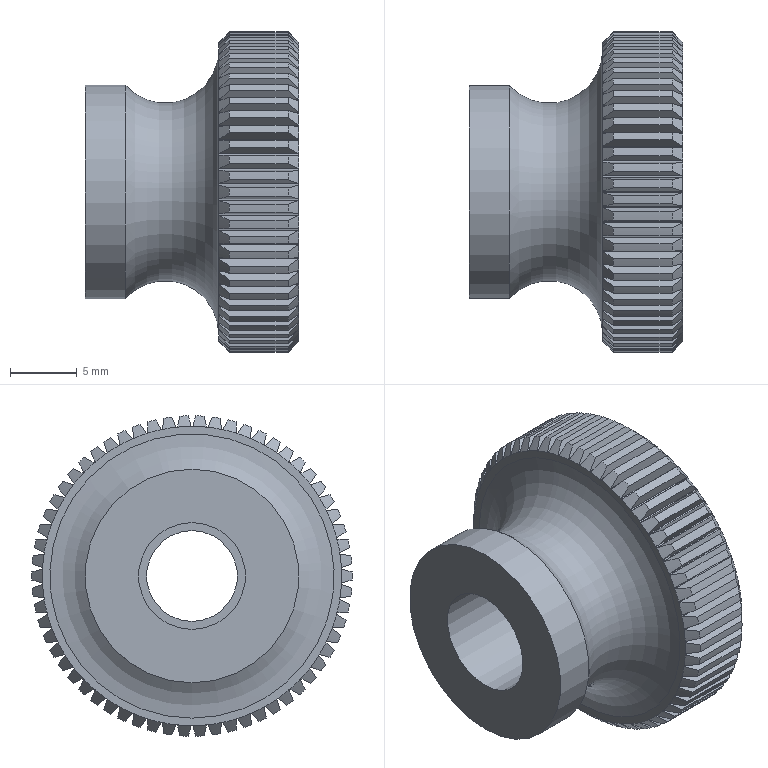Component | NX | HANDLE | 1 solid | 380 faces | volume 3652 mm3 | plane 190 | cone 124 | cylinder 65 | torus 1 | commonest cylinder face diameters 24 x62 16 x1 6.8 x1 8 x1